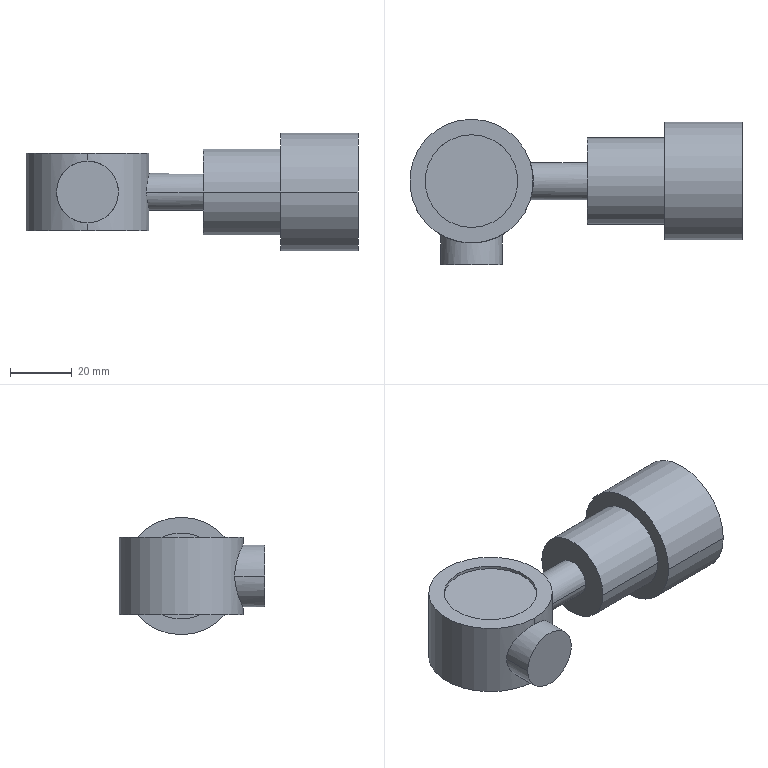Component | SolidWorks | InstrumentPanel-1 | 1 solid | 19 faces | box 107.5 x 47 x 38 mm | volume 78863 mm3 | cylinder 12 | plane 7 | commonest cylinder face diameters 30 x2 38 x2 28 x2 40 x2 20 x2 12 x2
build123d program:
from build123d import *

# Parameters (mm, degrees)
SKETCH1_R           = 10
BOSS_EXTRUDE1_DEPTH = 10
SKETCH2_R           = 20
BOSS_EXTRUDE2_DEPTH = 12.5
SKETCH3_W           = 6
SKETCH3_H           = 50
SKETCH4_R           = 14
BOSS_EXTRUDE3_DEPTH = 12.5
SKETCH5_R           = 19
BOSS_EXTRUDE4_DEPTH = 25
SKETCH6_R           = 15
CUT_EXTRUDE1_DEPTH  = 1


with BuildPart() as part:
    # Sketch1 → Boss-Extrude1 (new body)
    with BuildSketch(Plane.XY):
        with Locations((-171.265, 40.821)):
            Circle(SKETCH1_R)
    extrude(amount=BOSS_EXTRUDE1_DEPTH)

    # Sketch2 → Boss-Extrude2 (add, symmetric)
    with BuildSketch(Plane(origin=(0, 40.821, 0), x_dir=(0, 0, -1), z_dir=(0, -1, 0))):
        with Locations((-27, -171.265)):
            Circle(SKETCH2_R)
    extrude(amount=BOSS_EXTRUDE2_DEPTH, both=True)

    # Sketch3 → Revolve1 (revolve)
    with BuildSketch(Plane(origin=(0, 40.821, 0), x_dir=(0, 0, -1), z_dir=(0, -1, 0)), mode=Mode.PRIVATE) as revolve1_sk:
        with Locations((-24, -146.265)):
            Rectangle(SKETCH3_W, SKETCH3_H)
    revolve(revolve1_sk.sketch.rotate(Axis((-171.265, 40.821, 27), (1, 0, 0)), 180), axis=Axis((-171.265, 40.821, 27), (1, 0, 0)))

    # Sketch4 → Boss-Extrude3 (add, symmetric)
    with BuildSketch(Plane(origin=(-121.265, 0, 0), x_dir=(0, 0, -1), z_dir=(1, 0, 0))):
        with Locations((-27, 40.821)):
            Circle(SKETCH4_R)
    extrude(amount=BOSS_EXTRUDE3_DEPTH, both=True)

    # Sketch5 → Boss-Extrude4 (add)
    with BuildSketch(Plane(origin=(-108.765, 0, 0), x_dir=(0, 0, -1), z_dir=(1, 0, 0))):
        with Locations((-27, 40.821)):
            Circle(SKETCH5_R)
    extrude(amount=BOSS_EXTRUDE4_DEPTH)

    # Sketch6 → Cut-Extrude1 (cut, symmetric)
    with BuildSketch(Plane.XZ.offset(-28.321)):
        with Locations(Location((-171.265, 27, 0), (0, 0, 270))):
            Circle(SKETCH6_R)
    extrude(amount=CUT_EXTRUDE1_DEPTH, both=True, mode=Mode.SUBTRACT)


solid = part.part

# Placed as in the assembly
solid = solid.moved(Location((218.265, 195, 0.821), (-90, 0, 0)))
STEP:
#1=COLOUR_RGB('',0.7922,0.8196,0.9333);
#2=FILL_AREA_STYLE_COLOUR('',#1);
#3=FILL_AREA_STYLE('',(#2));
#4=SURFACE_STYLE_FILL_AREA(#3);
#5=SURFACE_SIDE_STYLE('',(#4));
#6=SURFACE_STYLE_USAGE(.BOTH.,#5);
#7=PRESENTATION_STYLE_ASSIGNMENT((#6));
#8=CARTESIAN_POINT('',(1.85,9.331,-1.122));
#9=VERTEX_POINT('',#8);
#10=CARTESIAN_POINT('',(1.85,8.15,-1.122));
#11=VERTEX_POINT('',#10);
#12=CARTESIAN_POINT('',(1.85,8.74,-1.122));
#13=DIRECTION('',(0.,0.,1.));
#14=DIRECTION('',(0.,-1.,0.));
#15=AXIS2_PLACEMENT_3D('',#12,#13,#14);
#16=CIRCLE('',#15,0.5906);
#17=EDGE_CURVE('',#9,#11,#16,.T.);
#18=ORIENTED_EDGE('',*,*,#17,.F.);
#19=CARTESIAN_POINT('',(1.85,9.331,-1.083));
#20=VERTEX_POINT('',#19);
#21=CARTESIAN_POINT('',(1.85,9.331,-1.122));
#22=DIRECTION('',(0.,0.,1.));
#23=VECTOR('',#22,39.37);
#24=LINE('',#21,#23);
#25=EDGE_CURVE('',#9,#20,#24,.T.);
#26=ORIENTED_EDGE('',*,*,#25,.T.);
#27=CARTESIAN_POINT('',(1.85,8.15,-1.083));
#28=VERTEX_POINT('',#27);
#29=CARTESIAN_POINT('',(1.85,8.74,-1.083));
#30=DIRECTION('',(0.,0.,1.));
#31=DIRECTION('',(0.,-1.,0.));
#32=AXIS2_PLACEMENT_3D('',#29,#30,#31);
#33=CIRCLE('',#32,0.5906);
#34=EDGE_CURVE('',#20,#28,#33,.T.);
#35=ORIENTED_EDGE('',*,*,#34,.T.);
#36=CARTESIAN_POINT('',(1.85,8.15,-1.122));
#37=DIRECTION('',(0.,0.,1.));
#38=VECTOR('',#37,39.37);
#39=LINE('',#36,#38);
#40=EDGE_CURVE('',#11,#28,#39,.T.);
#41=ORIENTED_EDGE('',*,*,#40,.F.);
#42=EDGE_LOOP('',(#18,#26,#35,#41));
#43=FACE_OUTER_BOUND('',#42,.T.);
#44=CARTESIAN_POINT('',(1.85,8.74,-1.122));
#45=DIRECTION('',(0.,0.,1.));
#46=DIRECTION('',(0.,-1.,0.));
#47=AXIS2_PLACEMENT_3D('',#44,#45,#46);
#48=CYLINDRICAL_SURFACE('',#47,0.5906);
#49=ADVANCED_FACE('',(#43),#48,.F.);
#50=CARTESIAN_POINT('',(5.295,7.992,-1.575));
#51=VERTEX_POINT('',#50);
#52=CARTESIAN_POINT('',(5.295,9.488,-1.575));
#53=VERTEX_POINT('',#52);
#54=CARTESIAN_POINT('',(5.295,8.74,-1.575));
#55=DIRECTION('',(1.,0.,0.));
#56=DIRECTION('',(0.,-1.,0.));
#57=AXIS2_PLACEMENT_3D('',#54,#55,#56);
#58=CIRCLE('',#57,0.748);
#59=EDGE_CURVE('',#51,#53,#58,.T.);
#60=ORIENTED_EDGE('',*,*,#59,.F.);
#61=CARTESIAN_POINT('',(4.311,7.992,-1.575));
#62=VERTEX_POINT('',#61);
#63=CARTESIAN_POINT('',(5.295,7.992,-1.575));
#64=DIRECTION('',(-1.,0.,0.));
#65=VECTOR('',#64,39.37);
#66=LINE('',#63,#65);
#67=EDGE_CURVE('',#51,#62,#66,.T.);
#68=ORIENTED_EDGE('',*,*,#67,.T.);
#69=CARTESIAN_POINT('',(4.311,9.488,-1.575));
#70=VERTEX_POINT('',#69);
#71=CARTESIAN_POINT('',(4.311,8.74,-1.575));
#72=DIRECTION('',(1.,0.,0.));
#73=DIRECTION('',(0.,-1.,0.));
#74=AXIS2_PLACEMENT_3D('',#71,#72,#73);
#75=CIRCLE('',#74,0.748);
#76=EDGE_CURVE('',#62,#70,#75,.T.);
#77=ORIENTED_EDGE('',*,*,#76,.T.);
#78=CARTESIAN_POINT('',(5.295,9.488,-1.575));
#79=DIRECTION('',(-1.,0.,0.));
#80=VECTOR('',#79,39.37);
#81=LINE('',#78,#80);
#82=EDGE_CURVE('',#53,#70,#81,.T.);
#83=ORIENTED_EDGE('',*,*,#82,.F.);
#84=EDGE_LOOP('',(#60,#68,#77,#83));
#85=FACE_OUTER_BOUND('',#84,.T.);
#86=CARTESIAN_POINT('',(5.295,8.74,-1.575));
#87=DIRECTION('',(-1.,0.,0.));
#88=DIRECTION('',(0.,1.,0.));
#89=AXIS2_PLACEMENT_3D('',#86,#87,#88);
#90=CYLINDRICAL_SURFACE('',#89,0.748);
#91=ADVANCED_FACE('',(#85),#90,.T.);
#92=CARTESIAN_POINT('',(4.311,8.189,-1.575));
#93=VERTEX_POINT('',#92);
#94=CARTESIAN_POINT('',(4.311,9.291,-1.575));
#95=VERTEX_POINT('',#94);
#96=CARTESIAN_POINT('',(4.311,8.74,-1.575));
#97=DIRECTION('',(1.,0.,0.));
#98=DIRECTION('',(0.,-1.,0.));
#99=AXIS2_PLACEMENT_3D('',#96,#97,#98);
#100=CIRCLE('',#99,0.5512);
#101=EDGE_CURVE('',#93,#95,#100,.T.);
#102=ORIENTED_EDGE('',*,*,#101,.F.);
#103=CARTESIAN_POINT('',(3.327,8.189,-1.575));
#104=VERTEX_POINT('',#103);
#105=CARTESIAN_POINT('',(4.311,8.189,-1.575));
#106=DIRECTION('',(-1.,0.,0.));
#107=VECTOR('',#106,39.37);
#108=LINE('',#105,#107);
#109=EDGE_CURVE('',#93,#104,#108,.T.);
#110=ORIENTED_EDGE('',*,*,#109,.T.);
#111=CARTESIAN_POINT('',(3.327,9.291,-1.575));
#112=VERTEX_POINT('',#111);
#113=CARTESIAN_POINT('',(3.327,8.74,-1.575));
#114=DIRECTION('',(1.,0.,0.));
#115=DIRECTION('',(0.,-1.,0.));
#116=AXIS2_PLACEMENT_3D('',#113,#114,#115);
#117=CIRCLE('',#116,0.5512);
#118=EDGE_CURVE('',#104,#112,#117,.T.);
#119=ORIENTED_EDGE('',*,*,#118,.T.);
#120=CARTESIAN_POINT('',(4.311,9.291,-1.575));
#121=DIRECTION('',(-1.,0.,0.));
#122=VECTOR('',#121,39.37);
#123=LINE('',#120,#122);
#124=EDGE_CURVE('',#95,#112,#123,.T.);
#125=ORIENTED_EDGE('',*,*,#124,.F.);
#126=EDGE_LOOP('',(#102,#110,#119,#125));
#127=FACE_OUTER_BOUND('',#126,.T.);
#128=CARTESIAN_POINT('',(4.311,8.74,-1.575));
#129=DIRECTION('',(-1.,0.,0.));
#130=DIRECTION('',(0.,1.,0.));
#131=AXIS2_PLACEMENT_3D('',#128,#129,#130);
#132=CYLINDRICAL_SURFACE('',#131,0.5512);
#133=ADVANCED_FACE('',(#127),#132,.T.);
#134=CARTESIAN_POINT('',(2.602,8.976,-1.575));
#135=VERTEX_POINT('',#134);
#136=CARTESIAN_POINT('',(2.602,8.504,-1.575));
#137=VERTEX_POINT('',#136);
#138=CARTESIAN_POINT('',(2.602,8.976,-1.575));
#139=CARTESIAN_POINT('',(2.602,8.976,-1.591));
#140=CARTESIAN_POINT('',(2.602,8.975,-1.606));
#141=CARTESIAN_POINT('',(2.603,8.97,-1.629));
#142=CARTESIAN_POINT('',(2.604,8.968,-1.636));
#143=CARTESIAN_POINT('',(2.605,8.964,-1.651));
#144=CARTESIAN_POINT('',(2.606,8.961,-1.658));
#145=CARTESIAN_POINT('',(2.609,8.952,-1.68));
#146=CARTESIAN_POINT('',(2.611,8.945,-1.693));
#147=CARTESIAN_POINT('',(2.614,8.932,-1.713));
#148=CARTESIAN_POINT('',(2.615,8.928,-1.719));
#149=CARTESIAN_POINT('',(2.618,8.918,-1.731));
#150=CARTESIAN_POINT('',(2.619,8.913,-1.736));
#151=CARTESIAN_POINT('',(2.622,8.896,-1.753));
#152=CARTESIAN_POINT('',(2.625,8.884,-1.762));
#153=CARTESIAN_POINT('',(2.629,8.859,-1.78));
#154=CARTESIAN_POINT('',(2.631,8.845,-1.787));
#155=CARTESIAN_POINT('',(2.633,8.824,-1.796));
#156=CARTESIAN_POINT('',(2.634,8.817,-1.798));
#157=CARTESIAN_POINT('',(2.635,8.802,-1.803));
#158=CARTESIAN_POINT('',(2.636,8.794,-1.805));
#159=CARTESIAN_POINT('',(2.637,8.771,-1.809));
#160=CARTESIAN_POINT('',(2.638,8.756,-1.811));
#161=CARTESIAN_POINT('',(2.638,8.725,-1.811));
#162=CARTESIAN_POINT('',(2.637,8.709,-1.809));
#163=CARTESIAN_POINT('',(2.636,8.679,-1.803));
#164=CARTESIAN_POINT('',(2.634,8.664,-1.799));
#165=CARTESIAN_POINT('',(2.631,8.635,-1.787));
#166=CARTESIAN_POINT('',(2.629,8.621,-1.78));
#167=CARTESIAN_POINT('',(2.626,8.602,-1.767));
#168=CARTESIAN_POINT('',(2.625,8.596,-1.762));
#169=CARTESIAN_POINT('',(2.622,8.584,-1.752));
#170=CARTESIAN_POINT('',(2.621,8.578,-1.747));
#171=CARTESIAN_POINT('',(2.617,8.562,-1.731));
#172=CARTESIAN_POINT('',(2.615,8.552,-1.719));
#173=CARTESIAN_POINT('',(2.611,8.535,-1.693));
#174=CARTESIAN_POINT('',(2.609,8.528,-1.68));
#175=CARTESIAN_POINT('',(2.605,8.516,-1.651));
#176=CARTESIAN_POINT('',(2.604,8.512,-1.636));
#177=CARTESIAN_POINT('',(2.602,8.507,-1.614));
#178=CARTESIAN_POINT('',(2.602,8.506,-1.606));
#179=CARTESIAN_POINT('',(2.602,8.504,-1.59));
#180=CARTESIAN_POINT('',(2.602,8.504,-1.583));
#181=CARTESIAN_POINT('',(2.602,8.504,-1.575));
#182=B_SPLINE_CURVE_WITH_KNOTS('',3,(#138,#139,#140,#141,#142,#143,#144,#145,#146,#147,#148,#149,#150,#151,#152,#153,#154,#155,#156,#157,#158,#159,#160,#161,#162,#163,#164,#165,#166,#167,#168,#169,#170,#171,#172,#173,#174,#175,#176,#177,#178,#179,#180,#181),.UNSPECIFIED.,.F.,.F.,(4,2,2,2,2,2,2,2,2,2,2,2,2,2,2,2,2,2,2,2,2,4),(0.,0.001179,0.001769,0.002358,0.003538,0.004127,0.004717,0.005896,0.007075,0.007665,0.008255,0.009434,0.01061,0.01179,0.01297,0.01356,0.01415,0.01533,0.01651,0.01769,0.01828,0.01887),.UNSPECIFIED.);
#183=EDGE_CURVE('',#135,#137,#182,.T.);
#184=ORIENTED_EDGE('',*,*,#183,.T.);
#185=CARTESIAN_POINT('',(2.602,8.504,-1.575));
#186=CARTESIAN_POINT('',(2.602,8.504,-1.559));
#187=CARTESIAN_POINT('',(2.602,8.505,-1.544));
#188=CARTESIAN_POINT('',(2.604,8.512,-1.513));
#189=CARTESIAN_POINT('',(2.605,8.516,-1.498));
#190=CARTESIAN_POINT('',(2.609,8.528,-1.47));
#191=CARTESIAN_POINT('',(2.611,8.535,-1.456));
#192=CARTESIAN_POINT('',(2.615,8.552,-1.431));
#193=CARTESIAN_POINT('',(2.617,8.562,-1.419));
#194=CARTESIAN_POINT('',(2.621,8.579,-1.402));
#195=CARTESIAN_POINT('',(2.622,8.584,-1.397));
#196=CARTESIAN_POINT('',(2.625,8.596,-1.387));
#197=CARTESIAN_POINT('',(2.626,8.602,-1.383));
#198=CARTESIAN_POINT('',(2.629,8.621,-1.37));
#199=CARTESIAN_POINT('',(2.631,8.635,-1.363));
#200=CARTESIAN_POINT('',(2.634,8.664,-1.351));
#201=CARTESIAN_POINT('',(2.636,8.679,-1.346));
#202=CARTESIAN_POINT('',(2.637,8.701,-1.342));
#203=CARTESIAN_POINT('',(2.637,8.709,-1.341));
#204=CARTESIAN_POINT('',(2.638,8.724,-1.339));
#205=CARTESIAN_POINT('',(2.638,8.732,-1.339));
#206=CARTESIAN_POINT('',(2.638,8.756,-1.339));
#207=CARTESIAN_POINT('',(2.637,8.771,-1.34));
#208=CARTESIAN_POINT('',(2.636,8.794,-1.345));
#209=CARTESIAN_POINT('',(2.635,8.802,-1.347));
#210=CARTESIAN_POINT('',(2.634,8.816,-1.351));
#211=CARTESIAN_POINT('',(2.633,8.824,-1.354));
#212=CARTESIAN_POINT('',(2.631,8.845,-1.363));
#213=CARTESIAN_POINT('',(2.629,8.859,-1.37));
#214=CARTESIAN_POINT('',(2.625,8.884,-1.387));
#215=CARTESIAN_POINT('',(2.622,8.896,-1.397));
#216=CARTESIAN_POINT('',(2.619,8.913,-1.413));
#217=CARTESIAN_POINT('',(2.618,8.918,-1.419));
#218=CARTESIAN_POINT('',(2.615,8.928,-1.431));
#219=CARTESIAN_POINT('',(2.614,8.932,-1.437));
#220=CARTESIAN_POINT('',(2.611,8.945,-1.456));
#221=CARTESIAN_POINT('',(2.609,8.952,-1.47));
#222=CARTESIAN_POINT('',(2.605,8.964,-1.498));
#223=CARTESIAN_POINT('',(2.604,8.969,-1.513));
#224=CARTESIAN_POINT('',(2.602,8.975,-1.544));
#225=CARTESIAN_POINT('',(2.602,8.976,-1.559));
#226=CARTESIAN_POINT('',(2.602,8.976,-1.575));
#227=B_SPLINE_CURVE_WITH_KNOTS('',3,(#185,#186,#187,#188,#189,#190,#191,#192,#193,#194,#195,#196,#197,#198,#199,#200,#201,#202,#203,#204,#205,#206,#207,#208,#209,#210,#211,#212,#213,#214,#215,#216,#217,#218,#219,#220,#221,#222,#223,#224,#225,#226),.UNSPECIFIED.,.F.,.F.,(4,2,2,2,2,2,2,2,2,2,2,2,2,2,2,2,2,2,2,2,4),(0.01887,0.02005,0.02123,0.0224,0.02358,0.02417,0.02476,0.02594,0.02712,0.02771,0.0283,0.02948,0.03007,0.03066,0.03184,0.03301,0.0336,0.03419,0.03537,0.03655,0.03773),.UNSPECIFIED.);
#228=EDGE_CURVE('',#137,#135,#227,.T.);
#229=ORIENTED_EDGE('',*,*,#228,.T.);
#230=EDGE_LOOP('',(#184,#229));
#231=FACE_BOUND('',#230,.T.);
#232=CARTESIAN_POINT('',(1.85,7.953,-1.083));
#233=VERTEX_POINT('',#232);
#234=CARTESIAN_POINT('',(1.85,9.528,-1.083));
#235=VERTEX_POINT('',#234);
#236=CARTESIAN_POINT('',(1.85,8.74,-1.083));
#237=DIRECTION('',(0.,0.,1.));
#238=DIRECTION('',(0.,-1.,0.));
#239=AXIS2_PLACEMENT_3D('',#236,#237,#238);
#240=CIRCLE('',#239,0.7874);
#241=EDGE_CURVE('',#233,#235,#240,.T.);
#242=ORIENTED_EDGE('',*,*,#241,.F.);
#243=CARTESIAN_POINT('',(1.85,7.953,-1.181));
#244=VERTEX_POINT('',#243);
#245=CARTESIAN_POINT('',(1.85,7.953,-1.083));
#246=DIRECTION('',(0.,0.,-1.));
#247=VECTOR('',#246,39.37);
#248=LINE('',#245,#247);
#249=EDGE_CURVE('',#233,#244,#248,.T.);
#250=ORIENTED_EDGE('',*,*,#249,.T.);
#251=CARTESIAN_POINT('',(2.244,8.058,-1.575));
#252=VERTEX_POINT('',#251);
#253=CARTESIAN_POINT('',(1.85,7.953,-1.181));
#254=CARTESIAN_POINT('',(1.864,7.953,-1.181));
#255=CARTESIAN_POINT('',(1.877,7.953,-1.182));
#256=CARTESIAN_POINT('',(1.903,7.954,-1.184));
#257=CARTESIAN_POINT('',(1.916,7.955,-1.186));
#258=CARTESIAN_POINT('',(1.941,7.958,-1.192));
#259=CARTESIAN_POINT('',(1.954,7.959,-1.195));
#260=CARTESIAN_POINT('',(1.979,7.963,-1.202));
#261=CARTESIAN_POINT('',(1.991,7.965,-1.207));
#262=CARTESIAN_POINT('',(2.027,7.972,-1.222));
#263=CARTESIAN_POINT('',(2.049,7.978,-1.234));
#264=CARTESIAN_POINT('',(2.081,7.987,-1.256));
#265=CARTESIAN_POINT('',(2.091,7.99,-1.263));
#266=CARTESIAN_POINT('',(2.111,7.997,-1.279));
#267=CARTESIAN_POINT('',(2.12,8.,-1.288));
#268=CARTESIAN_POINT('',(2.147,8.011,-1.315));
#269=CARTESIAN_POINT('',(2.163,8.017,-1.334));
#270=CARTESIAN_POINT('',(2.185,8.027,-1.366));
#271=CARTESIAN_POINT('',(2.191,8.03,-1.377));
#272=CARTESIAN_POINT('',(2.203,8.036,-1.4));
#273=CARTESIAN_POINT('',(2.209,8.039,-1.411));
#274=CARTESIAN_POINT('',(2.219,8.044,-1.435));
#275=CARTESIAN_POINT('',(2.223,8.046,-1.447));
#276=CARTESIAN_POINT('',(2.231,8.051,-1.472));
#277=CARTESIAN_POINT('',(2.234,8.052,-1.484));
#278=CARTESIAN_POINT('',(2.242,8.057,-1.523));
#279=CARTESIAN_POINT('',(2.244,8.058,-1.549));
#280=CARTESIAN_POINT('',(2.244,8.058,-1.575));
#281=B_SPLINE_CURVE_WITH_KNOTS('',3,(#253,#254,#255,#256,#257,#258,#259,#260,#261,#262,#263,#264,#265,#266,#267,#268,#269,#270,#271,#272,#273,#274,#275,#276,#277,#278,#279,#280),.UNSPECIFIED.,.F.,.F.,(4,2,2,2,2,2,2,2,2,2,2,2,2,4),(0.01591,0.0169,0.0179,0.01889,0.01988,0.02187,0.02286,0.02386,0.02584,0.02684,0.02783,0.02883,0.02982,0.03181),.UNSPECIFIED.);
#282=EDGE_CURVE('',#244,#252,#281,.T.);
#283=ORIENTED_EDGE('',*,*,#282,.T.);
#284=CARTESIAN_POINT('',(1.85,7.953,-1.969));
#285=VERTEX_POINT('',#284);
#286=CARTESIAN_POINT('',(2.244,8.058,-1.575));
#287=CARTESIAN_POINT('',(2.244,8.058,-1.588));
#288=CARTESIAN_POINT('',(2.243,8.058,-1.601));
#289=CARTESIAN_POINT('',(2.241,8.056,-1.627));
#290=CARTESIAN_POINT('',(2.239,8.055,-1.64));
#291=CARTESIAN_POINT('',(2.231,8.051,-1.678));
#292=CARTESIAN_POINT('',(2.223,8.047,-1.703));
#293=CARTESIAN_POINT('',(2.203,8.036,-1.751));
#294=CARTESIAN_POINT('',(2.191,8.03,-1.773));
#295=CARTESIAN_POINT('',(2.163,8.017,-1.816));
#296=CARTESIAN_POINT('',(2.147,8.01,-1.835));
#297=CARTESIAN_POINT('',(2.111,7.997,-1.871));
#298=CARTESIAN_POINT('',(2.091,7.99,-1.887));
#299=CARTESIAN_POINT('',(2.06,7.981,-1.909));
#300=CARTESIAN_POINT('',(2.048,7.978,-1.915));
#301=CARTESIAN_POINT('',(2.026,7.972,-1.927));
#302=CARTESIAN_POINT('',(2.014,7.97,-1.933));
#303=CARTESIAN_POINT('',(1.979,7.963,-1.948));
#304=CARTESIAN_POINT('',(1.954,7.959,-1.955));
#305=CARTESIAN_POINT('',(1.916,7.955,-1.963));
#306=CARTESIAN_POINT('',(1.902,7.954,-1.965));
#307=CARTESIAN_POINT('',(1.876,7.953,-1.968));
#308=CARTESIAN_POINT('',(1.863,7.953,-1.969));
#309=CARTESIAN_POINT('',(1.85,7.953,-1.969));
#310=B_SPLINE_CURVE_WITH_KNOTS('',3,(#286,#287,#288,#289,#290,#291,#292,#293,#294,#295,#296,#297,#298,#299,#300,#301,#302,#303,#304,#305,#306,#307,#308,#309),.UNSPECIFIED.,.F.,.F.,(4,2,2,2,2,2,2,2,2,2,2,4),(0.03181,0.0328,0.03379,0.03578,0.03776,0.03975,0.04173,0.04273,0.04372,0.0457,0.0467,0.04769),.UNSPECIFIED.);
#311=EDGE_CURVE('',#252,#285,#310,.T.);
#312=ORIENTED_EDGE('',*,*,#311,.T.);
#313=CARTESIAN_POINT('',(1.85,7.953,-2.067));
#314=VERTEX_POINT('',#313);
#315=CARTESIAN_POINT('',(1.85,7.953,-1.083));
#316=DIRECTION('',(0.,0.,-1.));
#317=VECTOR('',#316,39.37);
#318=LINE('',#315,#317);
#319=EDGE_CURVE('',#285,#314,#318,.T.);
#320=ORIENTED_EDGE('',*,*,#319,.T.);
#321=CARTESIAN_POINT('',(1.85,9.528,-2.067));
#322=VERTEX_POINT('',#321);
#323=CARTESIAN_POINT('',(1.85,8.74,-2.067));
#324=DIRECTION('',(0.,0.,1.));
#325=DIRECTION('',(0.,-1.,0.));
#326=AXIS2_PLACEMENT_3D('',#323,#324,#325);
#327=CIRCLE('',#326,0.7874);
#328=EDGE_CURVE('',#314,#322,#327,.T.);
#329=ORIENTED_EDGE('',*,*,#328,.T.);
#330=CARTESIAN_POINT('',(1.85,9.528,-1.083));
#331=DIRECTION('',(0.,0.,-1.));
#332=VECTOR('',#331,39.37);
#333=LINE('',#330,#332);
#334=EDGE_CURVE('',#235,#322,#333,.T.);
#335=ORIENTED_EDGE('',*,*,#334,.F.);
#336=EDGE_LOOP('',(#242,#250,#283,#312,#320,#329,#335));
#337=FACE_OUTER_BOUND('',#336,.T.);
#338=CARTESIAN_POINT('',(1.85,8.74,-1.083));
#339=DIRECTION('',(0.,0.,-1.));
#340=DIRECTION('',(0.,1.,0.));
#341=AXIS2_PLACEMENT_3D('',#338,#339,#340);
#342=CYLINDRICAL_SURFACE('',#341,0.7874);
#343=ADVANCED_FACE('',(#231,#337),#342,.T.);
#344=ORIENTED_EDGE('',*,*,#311,.F.);
#345=CARTESIAN_POINT('',(2.244,7.677,-1.575));
#346=VERTEX_POINT('',#345);
#347=CARTESIAN_POINT('',(2.244,8.071,-1.575));
#348=DIRECTION('',(0.,-1.,0.));
#349=VECTOR('',#348,39.37);
#350=LINE('',#347,#349);
#351=EDGE_CURVE('',#252,#346,#350,.T.);
#352=ORIENTED_EDGE('',*,*,#351,.T.);
#353=CARTESIAN_POINT('',(1.457,7.677,-1.575));
#354=VERTEX_POINT('',#353);
#355=CARTESIAN_POINT('',(1.85,7.677,-1.575));
#356=DIRECTION('',(0.,1.,0.));
#357=DIRECTION('',(1.,0.,0.));
#358=AXIS2_PLACEMENT_3D('',#355,#356,#357);
#359=CIRCLE('',#358,0.3937);
#360=EDGE_CURVE('',#346,#354,#359,.T.);
#361=ORIENTED_EDGE('',*,*,#360,.T.);
#362=CARTESIAN_POINT('',(1.457,8.058,-1.575));
#363=VERTEX_POINT('',#362);
#364=CARTESIAN_POINT('',(1.457,8.071,-1.575));
#365=DIRECTION('',(0.,-1.,0.));
#366=VECTOR('',#365,39.37);
#367=LINE('',#364,#366);
#368=EDGE_CURVE('',#363,#354,#367,.T.);
#369=ORIENTED_EDGE('',*,*,#368,.F.);
#370=CARTESIAN_POINT('',(1.85,7.953,-1.969));
#371=CARTESIAN_POINT('',(1.837,7.953,-1.969));
#372=CARTESIAN_POINT('',(1.824,7.953,-1.968));
#373=CARTESIAN_POINT('',(1.798,7.954,-1.965));
#374=CARTESIAN_POINT('',(1.785,7.955,-1.963));
#375=CARTESIAN_POINT('',(1.747,7.959,-1.955));
#376=CARTESIAN_POINT('',(1.722,7.963,-1.948));
#377=CARTESIAN_POINT('',(1.686,7.97,-1.933));
#378=CARTESIAN_POINT('',(1.674,7.973,-1.927));
#379=CARTESIAN_POINT('',(1.652,7.978,-1.915));
#380=CARTESIAN_POINT('',(1.641,7.981,-1.908));
#381=CARTESIAN_POINT('',(1.62,7.987,-1.894));
#382=CARTESIAN_POINT('',(1.61,7.99,-1.887));
#383=CARTESIAN_POINT('',(1.59,7.997,-1.87));
#384=CARTESIAN_POINT('',(1.581,8.,-1.862));
#385=CARTESIAN_POINT('',(1.554,8.011,-1.835));
#386=CARTESIAN_POINT('',(1.538,8.017,-1.815));
#387=CARTESIAN_POINT('',(1.517,8.027,-1.784));
#388=CARTESIAN_POINT('',(1.51,8.03,-1.773));
#389=CARTESIAN_POINT('',(1.498,8.036,-1.75));
#390=CARTESIAN_POINT('',(1.492,8.039,-1.739));
#391=CARTESIAN_POINT('',(1.477,8.047,-1.703));
#392=CARTESIAN_POINT('',(1.47,8.051,-1.679));
#393=CARTESIAN_POINT('',(1.462,8.055,-1.641));
#394=CARTESIAN_POINT('',(1.46,8.056,-1.628));
#395=CARTESIAN_POINT('',(1.457,8.058,-1.601));
#396=CARTESIAN_POINT('',(1.457,8.058,-1.588));
#397=CARTESIAN_POINT('',(1.457,8.058,-1.575));
#398=B_SPLINE_CURVE_WITH_KNOTS('',3,(#370,#371,#372,#373,#374,#375,#376,#377,#378,#379,#380,#381,#382,#383,#384,#385,#386,#387,#388,#389,#390,#391,#392,#393,#394,#395,#396,#397),.UNSPECIFIED.,.F.,.F.,(4,2,2,2,2,2,2,2,2,2,2,2,2,4),(0.04769,0.04868,0.04967,0.05166,0.05265,0.05364,0.05463,0.05562,0.05761,0.0586,0.05959,0.06157,0.06256,0.06356),.UNSPECIFIED.);
#399=EDGE_CURVE('',#285,#363,#398,.T.);
#400=ORIENTED_EDGE('',*,*,#399,.F.);
#401=EDGE_LOOP('',(#344,#352,#361,#369,#400));
#402=FACE_OUTER_BOUND('',#401,.T.);
#403=CARTESIAN_POINT('',(1.85,8.071,-1.575));
#404=DIRECTION('',(0.,-1.,0.));
#405=DIRECTION('',(-1.,0.,0.));
#406=AXIS2_PLACEMENT_3D('',#403,#404,#405);
#407=CYLINDRICAL_SURFACE('',#406,0.3937);
#408=ADVANCED_FACE('',(#402),#407,.T.);
#409=CARTESIAN_POINT('',(3.327,8.976,-1.575));
#410=VERTEX_POINT('',#409);
#411=CARTESIAN_POINT('',(3.327,8.504,-1.575));
#412=VERTEX_POINT('',#411);
#413=CARTESIAN_POINT('',(3.327,8.74,-1.575));
#414=DIRECTION('',(-1.,0.,0.));
#415=DIRECTION('',(0.,-1.,0.));
#416=AXIS2_PLACEMENT_3D('',#413,#414,#415);
#417=CIRCLE('',#416,0.2362);
#418=EDGE_CURVE('',#410,#412,#417,.T.);
#419=ORIENTED_EDGE('',*,*,#418,.T.);
#420=CARTESIAN_POINT('',(1.85,8.504,-1.575));
#421=DIRECTION('',(-1.,0.,0.));
#422=VECTOR('',#421,39.37);
#423=LINE('',#420,#422);
#424=EDGE_CURVE('',#412,#137,#423,.T.);
#425=ORIENTED_EDGE('',*,*,#424,.T.);
#426=ORIENTED_EDGE('',*,*,#183,.F.);
#427=CARTESIAN_POINT('',(1.85,8.976,-1.575));
#428=DIRECTION('',(-1.,0.,0.));
#429=VECTOR('',#428,39.37);
#430=LINE('',#427,#429);
#431=EDGE_CURVE('',#410,#135,#430,.T.);
#432=ORIENTED_EDGE('',*,*,#431,.F.);
#433=EDGE_LOOP('',(#419,#425,#426,#432));
#434=FACE_OUTER_BOUND('',#433,.T.);
#435=CARTESIAN_POINT('',(1.85,8.74,-1.575));
#436=DIRECTION('',(-1.,0.,0.));
#437=DIRECTION('',(0.,1.,0.));
#438=AXIS2_PLACEMENT_3D('',#435,#436,#437);
#439=CYLINDRICAL_SURFACE('',#438,0.2362);
#440=ADVANCED_FACE('',(#434),#439,.T.);
#441=ORIENTED_EDGE('',*,*,#424,.F.);
#442=CARTESIAN_POINT('',(3.327,8.74,-1.575));
#443=DIRECTION('',(-1.,0.,0.));
#444=DIRECTION('',(0.,-1.,0.));
#445=AXIS2_PLACEMENT_3D('',#442,#443,#444);
#446=CIRCLE('',#445,0.2362);
#447=EDGE_CURVE('',#412,#410,#446,.T.);
#448=ORIENTED_EDGE('',*,*,#447,.T.);
#449=ORIENTED_EDGE('',*,*,#431,.T.);
#450=ORIENTED_EDGE('',*,*,#228,.F.);
#451=EDGE_LOOP('',(#441,#448,#449,#450));
#452=FACE_OUTER_BOUND('',#451,.T.);
#453=CARTESIAN_POINT('',(1.85,8.74,-1.575));
#454=DIRECTION('',(-1.,0.,0.));
#455=DIRECTION('',(0.,1.,0.));
#456=AXIS2_PLACEMENT_3D('',#453,#454,#455);
#457=CYLINDRICAL_SURFACE('',#456,0.2362);
#458=ADVANCED_FACE('',(#452),#457,.T.);
#459=ORIENTED_EDGE('',*,*,#351,.F.);
#460=ORIENTED_EDGE('',*,*,#282,.F.);
#461=CARTESIAN_POINT('',(1.457,8.058,-1.575));
#462=CARTESIAN_POINT('',(1.457,8.058,-1.548));
#463=CARTESIAN_POINT('',(1.459,8.057,-1.522));
#464=CARTESIAN_POINT('',(1.467,8.052,-1.484));
#465=CARTESIAN_POINT('',(1.47,8.051,-1.472));
#466=CARTESIAN_POINT('',(1.478,8.046,-1.447));
#467=CARTESIAN_POINT('',(1.482,8.044,-1.434));
#468=CARTESIAN_POINT('',(1.497,8.036,-1.399));
#469=CARTESIAN_POINT('',(1.509,8.03,-1.376));
#470=CARTESIAN_POINT('',(1.531,8.02,-1.345));
#471=CARTESIAN_POINT('',(1.538,8.017,-1.334));
#472=CARTESIAN_POINT('',(1.555,8.01,-1.315));
#473=CARTESIAN_POINT('',(1.563,8.007,-1.305));
#474=CARTESIAN_POINT('',(1.581,8.,-1.288));
#475=CARTESIAN_POINT('',(1.59,7.997,-1.279));
#476=CARTESIAN_POINT('',(1.61,7.99,-1.263));
#477=CARTESIAN_POINT('',(1.62,7.987,-1.255));
#478=CARTESIAN_POINT('',(1.652,7.978,-1.234));
#479=CARTESIAN_POINT('',(1.675,7.972,-1.222));
#480=CARTESIAN_POINT('',(1.71,7.965,-1.207));
#481=CARTESIAN_POINT('',(1.722,7.963,-1.202));
#482=CARTESIAN_POINT('',(1.747,7.959,-1.195));
#483=CARTESIAN_POINT('',(1.76,7.958,-1.191));
#484=CARTESIAN_POINT('',(1.798,7.954,-1.184));
#485=CARTESIAN_POINT('',(1.824,7.953,-1.181));
#486=CARTESIAN_POINT('',(1.85,7.953,-1.181));
#487=B_SPLINE_CURVE_WITH_KNOTS('',3,(#461,#462,#463,#464,#465,#466,#467,#468,#469,#470,#471,#472,#473,#474,#475,#476,#477,#478,#479,#480,#481,#482,#483,#484,#485,#486),.UNSPECIFIED.,.F.,.F.,(4,2,2,2,2,2,2,2,2,2,2,2,4),(0.,0.001989,0.002983,0.003977,0.005966,0.00696,0.007955,0.008949,0.009943,0.01193,0.01293,0.01392,0.01591),.UNSPECIFIED.);
#488=EDGE_CURVE('',#363,#244,#487,.T.);
#489=ORIENTED_EDGE('',*,*,#488,.F.);
#490=ORIENTED_EDGE('',*,*,#368,.T.);
#491=CARTESIAN_POINT('',(1.85,7.677,-1.575));
#492=DIRECTION('',(0.,1.,0.));
#493=DIRECTION('',(1.,0.,0.));
#494=AXIS2_PLACEMENT_3D('',#491,#492,#493);
#495=CIRCLE('',#494,0.3937);
#496=EDGE_CURVE('',#354,#346,#495,.T.);
#497=ORIENTED_EDGE('',*,*,#496,.T.);
#498=EDGE_LOOP('',(#459,#460,#489,#490,#497));
#499=FACE_OUTER_BOUND('',#498,.T.);
#500=CARTESIAN_POINT('',(1.85,8.071,-1.575));
#501=DIRECTION('',(0.,-1.,0.));
#502=DIRECTION('',(-1.,0.,0.));
#503=AXIS2_PLACEMENT_3D('',#500,#501,#502);
#504=CYLINDRICAL_SURFACE('',#503,0.3937);
#505=ADVANCED_FACE('',(#499),#504,.T.);
#506=ORIENTED_EDGE('',*,*,#496,.F.);
#507=ORIENTED_EDGE('',*,*,#360,.F.);
#508=EDGE_LOOP('',(#506,#507));
#509=FACE_OUTER_BOUND('',#508,.T.);
#510=CARTESIAN_POINT('',(1.85,7.677,-1.575));
#511=DIRECTION('',(0.,1.,0.));
#512=DIRECTION('',(1.,0.,0.));
#513=AXIS2_PLACEMENT_3D('',#510,#511,#512);
#514=PLANE('',#513);
#515=ADVANCED_FACE('',(#509),#514,.F.);
#516=ORIENTED_EDGE('',*,*,#249,.F.);
#517=CARTESIAN_POINT('',(1.85,8.74,-1.083));
#518=DIRECTION('',(0.,0.,1.));
#519=DIRECTION('',(0.,-1.,0.));
#520=AXIS2_PLACEMENT_3D('',#517,#518,#519);
#521=CIRCLE('',#520,0.7874);
#522=EDGE_CURVE('',#235,#233,#521,.T.);
#523=ORIENTED_EDGE('',*,*,#522,.F.);
#524=ORIENTED_EDGE('',*,*,#334,.T.);
#525=CARTESIAN_POINT('',(1.85,8.74,-2.067));
#526=DIRECTION('',(0.,0.,1.));
#527=DIRECTION('',(0.,-1.,0.));
#528=AXIS2_PLACEMENT_3D('',#525,#526,#527);
#529=CIRCLE('',#528,0.7874);
#530=EDGE_CURVE('',#322,#314,#529,.T.);
#531=ORIENTED_EDGE('',*,*,#530,.T.);
#532=ORIENTED_EDGE('',*,*,#319,.F.);
#533=ORIENTED_EDGE('',*,*,#399,.T.);
#534=ORIENTED_EDGE('',*,*,#488,.T.);
#535=EDGE_LOOP('',(#516,#523,#524,#531,#532,#533,#534));
#536=FACE_OUTER_BOUND('',#535,.T.);
#537=CARTESIAN_POINT('',(1.85,8.74,-1.083));
#538=DIRECTION('',(0.,0.,-1.));
#539=DIRECTION('',(0.,1.,0.));
#540=AXIS2_PLACEMENT_3D('',#537,#538,#539);
#541=CYLINDRICAL_SURFACE('',#540,0.7874);
#542=ADVANCED_FACE('',(#536),#541,.T.);
#543=CARTESIAN_POINT('',(1.85,8.74,-1.083));
#544=DIRECTION('',(0.,0.,1.));
#545=DIRECTION('',(0.,-1.,0.));
#546=AXIS2_PLACEMENT_3D('',#543,#544,#545);
#547=CIRCLE('',#546,0.5906);
#548=EDGE_CURVE('',#28,#20,#547,.T.);
#549=ORIENTED_EDGE('',*,*,#548,.F.);
#550=ORIENTED_EDGE('',*,*,#34,.F.);
#551=EDGE_LOOP('',(#549,#550));
#552=FACE_BOUND('',#551,.T.);
#553=ORIENTED_EDGE('',*,*,#522,.T.);
#554=ORIENTED_EDGE('',*,*,#241,.T.);
#555=EDGE_LOOP('',(#553,#554));
#556=FACE_OUTER_BOUND('',#555,.T.);
#557=CARTESIAN_POINT('',(1.85,8.74,-1.083));
#558=DIRECTION('',(0.,0.,1.));
#559=DIRECTION('',(0.,-1.,0.));
#560=AXIS2_PLACEMENT_3D('',#557,#558,#559);
#561=PLANE('',#560);
#562=ADVANCED_FACE('',(#552,#556),#561,.T.);
#563=ORIENTED_EDGE('',*,*,#530,.F.);
#564=ORIENTED_EDGE('',*,*,#328,.F.);
#565=EDGE_LOOP('',(#563,#564));
#566=FACE_OUTER_BOUND('',#565,.T.);
#567=CARTESIAN_POINT('',(1.85,8.74,-2.067));
#568=DIRECTION('',(0.,0.,1.));
#569=DIRECTION('',(0.,-1.,0.));
#570=AXIS2_PLACEMENT_3D('',#567,#568,#569);
#571=PLANE('',#570);
#572=ADVANCED_FACE('',(#566),#571,.F.);
#573=ORIENTED_EDGE('',*,*,#109,.F.);
#574=CARTESIAN_POINT('',(4.311,8.74,-1.575));
#575=DIRECTION('',(1.,0.,0.));
#576=DIRECTION('',(0.,-1.,0.));
#577=AXIS2_PLACEMENT_3D('',#574,#575,#576);
#578=CIRCLE('',#577,0.5512);
#579=EDGE_CURVE('',#95,#93,#578,.T.);
#580=ORIENTED_EDGE('',*,*,#579,.F.);
#581=ORIENTED_EDGE('',*,*,#124,.T.);
#582=CARTESIAN_POINT('',(3.327,8.74,-1.575));
#583=DIRECTION('',(1.,0.,0.));
#584=DIRECTION('',(0.,-1.,0.));
#585=AXIS2_PLACEMENT_3D('',#582,#583,#584);
#586=CIRCLE('',#585,0.5512);
#587=EDGE_CURVE('',#112,#104,#586,.T.);
#588=ORIENTED_EDGE('',*,*,#587,.T.);
#589=EDGE_LOOP('',(#573,#580,#581,#588));
#590=FACE_OUTER_BOUND('',#589,.T.);
#591=CARTESIAN_POINT('',(4.311,8.74,-1.575));
#592=DIRECTION('',(-1.,0.,0.));
#593=DIRECTION('',(0.,1.,0.));
#594=AXIS2_PLACEMENT_3D('',#591,#592,#593);
#595=CYLINDRICAL_SURFACE('',#594,0.5512);
#596=ADVANCED_FACE('',(#590),#595,.T.);
#597=ORIENTED_EDGE('',*,*,#418,.F.);
#598=ORIENTED_EDGE('',*,*,#447,.F.);
#599=EDGE_LOOP('',(#597,#598));
#600=FACE_BOUND('',#599,.T.);
#601=ORIENTED_EDGE('',*,*,#587,.F.);
#602=ORIENTED_EDGE('',*,*,#118,.F.);
#603=EDGE_LOOP('',(#601,#602));
#604=FACE_OUTER_BOUND('',#603,.T.);
#605=CARTESIAN_POINT('',(3.327,8.74,-1.575));
#606=DIRECTION('',(1.,0.,0.));
#607=DIRECTION('',(0.,-1.,0.));
#608=AXIS2_PLACEMENT_3D('',#605,#606,#607);
#609=PLANE('',#608);
#610=ADVANCED_FACE('',(#600,#604),#609,.F.);
#611=ORIENTED_EDGE('',*,*,#67,.F.);
#612=CARTESIAN_POINT('',(5.295,8.74,-1.575));
#613=DIRECTION('',(1.,0.,0.));
#614=DIRECTION('',(0.,-1.,0.));
#615=AXIS2_PLACEMENT_3D('',#612,#613,#614);
#616=CIRCLE('',#615,0.748);
#617=EDGE_CURVE('',#53,#51,#616,.T.);
#618=ORIENTED_EDGE('',*,*,#617,.F.);
#619=ORIENTED_EDGE('',*,*,#82,.T.);
#620=CARTESIAN_POINT('',(4.311,8.74,-1.575));
#621=DIRECTION('',(1.,0.,0.));
#622=DIRECTION('',(0.,-1.,0.));
#623=AXIS2_PLACEMENT_3D('',#620,#621,#622);
#624=CIRCLE('',#623,0.748);
#625=EDGE_CURVE('',#70,#62,#624,.T.);
#626=ORIENTED_EDGE('',*,*,#625,.T.);
#627=EDGE_LOOP('',(#611,#618,#619,#626));
#628=FACE_OUTER_BOUND('',#627,.T.);
#629=CARTESIAN_POINT('',(5.295,8.74,-1.575));
#630=DIRECTION('',(-1.,0.,0.));
#631=DIRECTION('',(0.,1.,0.));
#632=AXIS2_PLACEMENT_3D('',#629,#630,#631);
#633=CYLINDRICAL_SURFACE('',#632,0.748);
#634=ADVANCED_FACE('',(#628),#633,.T.);
#635=ORIENTED_EDGE('',*,*,#617,.T.);
#636=ORIENTED_EDGE('',*,*,#59,.T.);
#637=EDGE_LOOP('',(#635,#636));
#638=FACE_OUTER_BOUND('',#637,.T.);
#639=CARTESIAN_POINT('',(5.295,8.74,-1.575));
#640=DIRECTION('',(1.,0.,0.));
#641=DIRECTION('',(0.,-1.,0.));
#642=AXIS2_PLACEMENT_3D('',#639,#640,#641);
#643=PLANE('',#642);
#644=ADVANCED_FACE('',(#638),#643,.T.);
#645=ORIENTED_EDGE('',*,*,#579,.T.);
#646=ORIENTED_EDGE('',*,*,#101,.T.);
#647=EDGE_LOOP('',(#645,#646));
#648=FACE_BOUND('',#647,.T.);
#649=ORIENTED_EDGE('',*,*,#625,.F.);
#650=ORIENTED_EDGE('',*,*,#76,.F.);
#651=EDGE_LOOP('',(#649,#650));
#652=FACE_OUTER_BOUND('',#651,.T.);
#653=CARTESIAN_POINT('',(4.311,8.74,-1.575));
#654=DIRECTION('',(1.,0.,0.));
#655=DIRECTION('',(0.,-1.,0.));
#656=AXIS2_PLACEMENT_3D('',#653,#654,#655);
#657=PLANE('',#656);
#658=ADVANCED_FACE('',(#648,#652),#657,.F.);
#659=ORIENTED_EDGE('',*,*,#25,.F.);
#660=CARTESIAN_POINT('',(1.85,8.74,-1.122));
#661=DIRECTION('',(0.,0.,1.));
#662=DIRECTION('',(0.,-1.,0.));
#663=AXIS2_PLACEMENT_3D('',#660,#661,#662);
#664=CIRCLE('',#663,0.5906);
#665=EDGE_CURVE('',#11,#9,#664,.T.);
#666=ORIENTED_EDGE('',*,*,#665,.F.);
#667=ORIENTED_EDGE('',*,*,#40,.T.);
#668=ORIENTED_EDGE('',*,*,#548,.T.);
#669=EDGE_LOOP('',(#659,#666,#667,#668));
#670=FACE_OUTER_BOUND('',#669,.T.);
#671=CARTESIAN_POINT('',(1.85,8.74,-1.122));
#672=DIRECTION('',(0.,0.,1.));
#673=DIRECTION('',(0.,-1.,0.));
#674=AXIS2_PLACEMENT_3D('',#671,#672,#673);
#675=CYLINDRICAL_SURFACE('',#674,0.5906);
#676=ADVANCED_FACE('',(#670),#675,.F.);
#677=ORIENTED_EDGE('',*,*,#665,.T.);
#678=ORIENTED_EDGE('',*,*,#17,.T.);
#679=EDGE_LOOP('',(#677,#678));
#680=FACE_OUTER_BOUND('',#679,.T.);
#681=CARTESIAN_POINT('',(1.85,8.74,-1.122));
#682=DIRECTION('',(0.,0.,1.));
#683=DIRECTION('',(0.,-1.,0.));
#684=AXIS2_PLACEMENT_3D('',#681,#682,#683);
#685=PLANE('',#684);
#686=ADVANCED_FACE('',(#680),#685,.T.);
#687=CLOSED_SHELL('',(#49,#91,#133,#343,#408,#440,#458,#505,#515,#542,#562,#572,#596,#610,#634,#644,#658,#676,#686));
#688=MANIFOLD_SOLID_BREP('',#687);
#689=STYLED_ITEM('',(#7),#688);
#690=(LENGTH_UNIT()NAMED_UNIT(*)SI_UNIT($,.METRE.));
#691=LENGTH_MEASURE_WITH_UNIT(LENGTH_MEASURE(0.0254),#690);
#692=DIMENSIONAL_EXPONENTS(1.,0.,0.,0.,0.,0.,0.);
#693=(CONVERSION_BASED_UNIT('',#691)LENGTH_UNIT()NAMED_UNIT(#692));
#694=UNCERTAINTY_MEASURE_WITH_UNIT(LENGTH_MEASURE(0.00001),#693,'','');
#695=(NAMED_UNIT(*)PLANE_ANGLE_UNIT()SI_UNIT($,.RADIAN.));
#696=(NAMED_UNIT(*)SI_UNIT($,.STERADIAN.)SOLID_ANGLE_UNIT());
#697=(GEOMETRIC_REPRESENTATION_CONTEXT(3)GLOBAL_UNCERTAINTY_ASSIGNED_CONTEXT((#694))GLOBAL_UNIT_ASSIGNED_CONTEXT((#693,#695,#696))REPRESENTATION_CONTEXT('',''));
#698=MECHANICAL_DESIGN_GEOMETRIC_PRESENTATION_REPRESENTATION('',(#689),#697);
#699=CARTESIAN_POINT('',(0.,0.,0.));
#700=DIRECTION('',(0.,0.,1.));
#701=DIRECTION('',(1.,0.,0.));
#702=AXIS2_PLACEMENT_3D('',#699,#700,#701);
#703=(LENGTH_UNIT()NAMED_UNIT(*)SI_UNIT($,.METRE.));
#704=LENGTH_MEASURE_WITH_UNIT(LENGTH_MEASURE(0.0254),#703);
#705=DIMENSIONAL_EXPONENTS(1.,0.,0.,0.,0.,0.,0.);
#706=(CONVERSION_BASED_UNIT('',#704)LENGTH_UNIT()NAMED_UNIT(#705));
#707=UNCERTAINTY_MEASURE_WITH_UNIT(LENGTH_MEASURE(0.00001),#706,'','');
#708=(NAMED_UNIT(*)PLANE_ANGLE_UNIT()SI_UNIT($,.RADIAN.));
#709=(NAMED_UNIT(*)SI_UNIT($,.STERADIAN.)SOLID_ANGLE_UNIT());
#710=(GEOMETRIC_REPRESENTATION_CONTEXT(3)GLOBAL_UNCERTAINTY_ASSIGNED_CONTEXT((#707))GLOBAL_UNIT_ASSIGNED_CONTEXT((#706,#708,#709))REPRESENTATION_CONTEXT('',''));
#711=ADVANCED_BREP_SHAPE_REPRESENTATION('',(#688,#702),#710);
#712=PRESENTATION_LAYER_ASSIGNMENT('','',(#689));